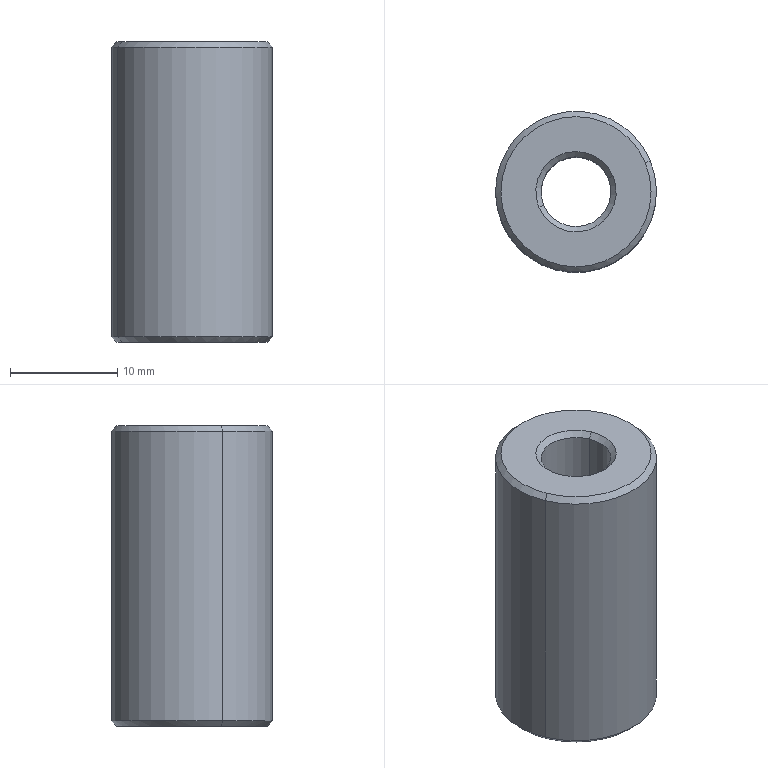Component | SolidWorks | WT-FLD-EJG-1212-00-024-1 | 1 solid | 14 faces | box 15 x 15 x 28 mm | volume 4002 mm3 | cone 8 | cylinder 4 | plane 2 | commonest cylinder face diameters 6.5 x2 15 x2 | material AISI 1045 Steel, cold drawn
build123d program:
from build123d import *

# Parameters (mm, degrees)
SKETCH1_R                  = 7.5
BOSS_EXTRUDE1_DEPTH        = 28
F_6_5_6_5_DIAMETER_HOLE1_D = 6.5
CHAMFER1_SIZE              = 0.5


with BuildPart() as part:
    # Sketch1 → Boss-Extrude1 (new body)
    with BuildSketch(Plane.XY):
        Circle(SKETCH1_R)
    extrude(amount=BOSS_EXTRUDE1_DEPTH)

    # 6.5 _6.5_ Diameter Hole1 (through all)
    with Locations(Plane.XY.offset(28)):
        with Locations((0, 0)):
            Hole(F_6_5_6_5_DIAMETER_HOLE1_D / 2)

    # Chamfer1
    chamfer1_edges = [part.edges().sort_by_distance(p)[0] for p in [
        (-7.5, 0, 0),
        (-7.5, 0, 28),
        (3.25, 0, 28),
        (3.25, 0, 0),
    ]]
    chamfer(chamfer1_edges, length=CHAMFER1_SIZE)


solid = part.part

# Placed as in the assembly
solid = solid.moved(Location((-97, -50, 60), (0, 0, 0)))
STEP:
#1=COLOUR_RGB('',0.7922,0.8196,0.9333);
#2=FILL_AREA_STYLE_COLOUR('',#1);
#3=FILL_AREA_STYLE('',(#2));
#4=SURFACE_STYLE_FILL_AREA(#3);
#5=SURFACE_SIDE_STYLE('',(#4));
#6=SURFACE_STYLE_USAGE(.BOTH.,#5);
#7=PRESENTATION_STYLE_ASSIGNMENT((#6));
#8=CARTESIAN_POINT('',(-3.701,-1.919,2.382));
#9=VERTEX_POINT('',#8);
#10=CARTESIAN_POINT('',(-3.937,-2.018,2.382));
#11=VERTEX_POINT('',#10);
#12=CARTESIAN_POINT('',(-3.819,-1.969,2.382));
#13=DIRECTION('',(0.,-0.,-1.));
#14=DIRECTION('',(-0.9237,-0.383,0.));
#15=AXIS2_PLACEMENT_3D('',#12,#13,#14);
#16=CIRCLE('',#15,0.128);
#17=EDGE_CURVE('',#9,#11,#16,.T.);
#18=ORIENTED_EDGE('',*,*,#17,.F.);
#19=CARTESIAN_POINT('',(-3.683,-1.912,2.362));
#20=VERTEX_POINT('',#19);
#21=CARTESIAN_POINT('',(-3.701,-1.919,2.382));
#22=DIRECTION('',(0.6532,0.2709,-0.7071));
#23=VECTOR('',#22,39.37);
#24=LINE('',#21,#23);
#25=EDGE_CURVE('',#9,#20,#24,.T.);
#26=ORIENTED_EDGE('',*,*,#25,.T.);
#27=CARTESIAN_POINT('',(-3.955,-2.025,2.362));
#28=VERTEX_POINT('',#27);
#29=CARTESIAN_POINT('',(-3.819,-1.969,2.362));
#30=DIRECTION('',(-0.,0.,1.));
#31=DIRECTION('',(-0.9237,-0.383,0.));
#32=AXIS2_PLACEMENT_3D('',#29,#30,#31);
#33=CIRCLE('',#32,0.1476);
#34=EDGE_CURVE('',#28,#20,#33,.T.);
#35=ORIENTED_EDGE('',*,*,#34,.F.);
#36=CARTESIAN_POINT('',(-3.937,-2.018,2.382));
#37=DIRECTION('',(-0.6532,-0.2709,-0.7071));
#38=VECTOR('',#37,39.37);
#39=LINE('',#36,#38);
#40=EDGE_CURVE('',#11,#28,#39,.T.);
#41=ORIENTED_EDGE('',*,*,#40,.F.);
#42=EDGE_LOOP('',(#18,#26,#35,#41));
#43=FACE_OUTER_BOUND('',#42,.T.);
#44=CARTESIAN_POINT('',(-3.819,-1.969,2.382));
#45=DIRECTION('',(0.,-0.,-1.));
#46=DIRECTION('',(-0.9237,-0.383,0.));
#47=AXIS2_PLACEMENT_3D('',#44,#45,#46);
#48=CONICAL_SURFACE('',#47,0.128,0.7854);
#49=ADVANCED_FACE('',(#43),#48,.F.);
#50=CARTESIAN_POINT('',(-4.073,-2.074,2.362));
#51=VERTEX_POINT('',#50);
#52=CARTESIAN_POINT('',(-3.564,-1.863,2.362));
#53=VERTEX_POINT('',#52);
#54=CARTESIAN_POINT('',(-3.819,-1.969,2.362));
#55=DIRECTION('',(0.,-0.,-1.));
#56=DIRECTION('',(-0.9237,-0.383,0.));
#57=AXIS2_PLACEMENT_3D('',#54,#55,#56);
#58=CIRCLE('',#57,0.2756);
#59=EDGE_CURVE('',#51,#53,#58,.T.);
#60=ORIENTED_EDGE('',*,*,#59,.F.);
#61=CARTESIAN_POINT('',(-4.092,-2.082,2.382));
#62=VERTEX_POINT('',#61);
#63=CARTESIAN_POINT('',(-4.073,-2.074,2.362));
#64=DIRECTION('',(-0.6532,-0.2709,0.7071));
#65=VECTOR('',#64,39.37);
#66=LINE('',#63,#65);
#67=EDGE_CURVE('',#51,#62,#66,.T.);
#68=ORIENTED_EDGE('',*,*,#67,.T.);
#69=CARTESIAN_POINT('',(-3.546,-1.855,2.382));
#70=VERTEX_POINT('',#69);
#71=CARTESIAN_POINT('',(-3.819,-1.969,2.382));
#72=DIRECTION('',(-0.,0.,1.));
#73=DIRECTION('',(-0.9237,-0.383,0.));
#74=AXIS2_PLACEMENT_3D('',#71,#72,#73);
#75=CIRCLE('',#74,0.2953);
#76=EDGE_CURVE('',#70,#62,#75,.T.);
#77=ORIENTED_EDGE('',*,*,#76,.F.);
#78=CARTESIAN_POINT('',(-3.564,-1.863,2.362));
#79=DIRECTION('',(0.6532,0.2709,0.7071));
#80=VECTOR('',#79,39.37);
#81=LINE('',#78,#80);
#82=EDGE_CURVE('',#53,#70,#81,.T.);
#83=ORIENTED_EDGE('',*,*,#82,.F.);
#84=EDGE_LOOP('',(#60,#68,#77,#83));
#85=FACE_OUTER_BOUND('',#84,.T.);
#86=CARTESIAN_POINT('',(-3.819,-1.969,2.362));
#87=DIRECTION('',(-0.,0.,1.));
#88=DIRECTION('',(0.9237,0.383,-0.));
#89=AXIS2_PLACEMENT_3D('',#86,#87,#88);
#90=CONICAL_SURFACE('',#89,0.2756,0.7854);
#91=ADVANCED_FACE('',(#85),#90,.T.);
#92=CARTESIAN_POINT('',(-3.937,-2.018,3.445));
#93=VERTEX_POINT('',#92);
#94=CARTESIAN_POINT('',(-3.701,-1.919,3.445));
#95=VERTEX_POINT('',#94);
#96=CARTESIAN_POINT('',(-3.819,-1.969,3.445));
#97=DIRECTION('',(-0.,0.,1.));
#98=DIRECTION('',(-0.9237,-0.383,0.));
#99=AXIS2_PLACEMENT_3D('',#96,#97,#98);
#100=CIRCLE('',#99,0.128);
#101=EDGE_CURVE('',#93,#95,#100,.T.);
#102=ORIENTED_EDGE('',*,*,#101,.F.);
#103=CARTESIAN_POINT('',(-3.955,-2.025,3.465));
#104=VERTEX_POINT('',#103);
#105=CARTESIAN_POINT('',(-3.955,-2.025,3.465));
#106=DIRECTION('',(-0.6532,-0.2709,0.7071));
#107=VECTOR('',#106,39.37);
#108=LINE('',#105,#107);
#109=EDGE_CURVE('',#93,#104,#108,.T.);
#110=ORIENTED_EDGE('',*,*,#109,.T.);
#111=CARTESIAN_POINT('',(-3.683,-1.912,3.465));
#112=VERTEX_POINT('',#111);
#113=CARTESIAN_POINT('',(-3.819,-1.969,3.465));
#114=DIRECTION('',(0.,-0.,-1.));
#115=DIRECTION('',(-0.9237,-0.383,0.));
#116=AXIS2_PLACEMENT_3D('',#113,#114,#115);
#117=CIRCLE('',#116,0.1476);
#118=EDGE_CURVE('',#112,#104,#117,.T.);
#119=ORIENTED_EDGE('',*,*,#118,.F.);
#120=CARTESIAN_POINT('',(-3.683,-1.912,3.465));
#121=DIRECTION('',(0.6532,0.2709,0.7071));
#122=VECTOR('',#121,39.37);
#123=LINE('',#120,#122);
#124=EDGE_CURVE('',#95,#112,#123,.T.);
#125=ORIENTED_EDGE('',*,*,#124,.F.);
#126=EDGE_LOOP('',(#102,#110,#119,#125));
#127=FACE_OUTER_BOUND('',#126,.T.);
#128=CARTESIAN_POINT('',(-3.819,-1.969,3.465));
#129=DIRECTION('',(-0.,0.,1.));
#130=DIRECTION('',(0.9237,0.383,0.));
#131=AXIS2_PLACEMENT_3D('',#128,#129,#130);
#132=CONICAL_SURFACE('',#131,0.1476,0.7854);
#133=ADVANCED_FACE('',(#127),#132,.F.);
#134=CARTESIAN_POINT('',(-3.564,-1.863,3.465));
#135=VERTEX_POINT('',#134);
#136=CARTESIAN_POINT('',(-4.073,-2.074,3.465));
#137=VERTEX_POINT('',#136);
#138=CARTESIAN_POINT('',(-3.819,-1.969,3.465));
#139=DIRECTION('',(-0.,0.,1.));
#140=DIRECTION('',(-0.9237,-0.383,0.));
#141=AXIS2_PLACEMENT_3D('',#138,#139,#140);
#142=CIRCLE('',#141,0.2756);
#143=EDGE_CURVE('',#135,#137,#142,.T.);
#144=ORIENTED_EDGE('',*,*,#143,.F.);
#145=CARTESIAN_POINT('',(-3.546,-1.855,3.445));
#146=VERTEX_POINT('',#145);
#147=CARTESIAN_POINT('',(-3.546,-1.855,3.445));
#148=DIRECTION('',(0.6532,0.2709,-0.7071));
#149=VECTOR('',#148,39.37);
#150=LINE('',#147,#149);
#151=EDGE_CURVE('',#135,#146,#150,.T.);
#152=ORIENTED_EDGE('',*,*,#151,.T.);
#153=CARTESIAN_POINT('',(-4.092,-2.082,3.445));
#154=VERTEX_POINT('',#153);
#155=CARTESIAN_POINT('',(-3.819,-1.969,3.445));
#156=DIRECTION('',(0.,-0.,-1.));
#157=DIRECTION('',(-0.9237,-0.383,0.));
#158=AXIS2_PLACEMENT_3D('',#155,#156,#157);
#159=CIRCLE('',#158,0.2953);
#160=EDGE_CURVE('',#154,#146,#159,.T.);
#161=ORIENTED_EDGE('',*,*,#160,.F.);
#162=CARTESIAN_POINT('',(-4.092,-2.082,3.445));
#163=DIRECTION('',(-0.6532,-0.2709,-0.7071));
#164=VECTOR('',#163,39.37);
#165=LINE('',#162,#164);
#166=EDGE_CURVE('',#137,#154,#165,.T.);
#167=ORIENTED_EDGE('',*,*,#166,.F.);
#168=EDGE_LOOP('',(#144,#152,#161,#167));
#169=FACE_OUTER_BOUND('',#168,.T.);
#170=CARTESIAN_POINT('',(-3.819,-1.969,3.445));
#171=DIRECTION('',(0.,-0.,-1.));
#172=DIRECTION('',(-0.9237,-0.383,0.));
#173=AXIS2_PLACEMENT_3D('',#170,#171,#172);
#174=CONICAL_SURFACE('',#173,0.2953,0.7854);
#175=ADVANCED_FACE('',(#169),#174,.T.);
#176=ORIENTED_EDGE('',*,*,#101,.T.);
#177=CARTESIAN_POINT('',(-3.701,-1.919,2.362));
#178=DIRECTION('',(0.,-0.,-1.));
#179=VECTOR('',#178,39.37);
#180=LINE('',#177,#179);
#181=EDGE_CURVE('',#95,#9,#180,.T.);
#182=ORIENTED_EDGE('',*,*,#181,.T.);
#183=ORIENTED_EDGE('',*,*,#17,.T.);
#184=CARTESIAN_POINT('',(-3.937,-2.018,2.362));
#185=DIRECTION('',(0.,-0.,-1.));
#186=VECTOR('',#185,39.37);
#187=LINE('',#184,#186);
#188=EDGE_CURVE('',#93,#11,#187,.T.);
#189=ORIENTED_EDGE('',*,*,#188,.F.);
#190=EDGE_LOOP('',(#176,#182,#183,#189));
#191=FACE_OUTER_BOUND('',#190,.T.);
#192=CARTESIAN_POINT('',(-3.819,-1.969,2.362));
#193=DIRECTION('',(0.,-0.,-1.));
#194=DIRECTION('',(-0.9237,-0.383,0.));
#195=AXIS2_PLACEMENT_3D('',#192,#193,#194);
#196=CYLINDRICAL_SURFACE('',#195,0.128);
#197=ADVANCED_FACE('',(#191),#196,.F.);
#198=ORIENTED_EDGE('',*,*,#76,.T.);
#199=CARTESIAN_POINT('',(-4.092,-2.082,2.362));
#200=DIRECTION('',(-0.,0.,1.));
#201=VECTOR('',#200,39.37);
#202=LINE('',#199,#201);
#203=EDGE_CURVE('',#62,#154,#202,.T.);
#204=ORIENTED_EDGE('',*,*,#203,.T.);
#205=ORIENTED_EDGE('',*,*,#160,.T.);
#206=CARTESIAN_POINT('',(-3.546,-1.855,2.362));
#207=DIRECTION('',(-0.,0.,1.));
#208=VECTOR('',#207,39.37);
#209=LINE('',#206,#208);
#210=EDGE_CURVE('',#70,#146,#209,.T.);
#211=ORIENTED_EDGE('',*,*,#210,.F.);
#212=EDGE_LOOP('',(#198,#204,#205,#211));
#213=FACE_OUTER_BOUND('',#212,.T.);
#214=CARTESIAN_POINT('',(-3.819,-1.969,2.362));
#215=DIRECTION('',(-0.,0.,1.));
#216=DIRECTION('',(0.9237,0.383,-0.));
#217=AXIS2_PLACEMENT_3D('',#214,#215,#216);
#218=CYLINDRICAL_SURFACE('',#217,0.2953);
#219=ADVANCED_FACE('',(#213),#218,.T.);
#220=ORIENTED_EDGE('',*,*,#203,.F.);
#221=CARTESIAN_POINT('',(-3.819,-1.969,2.382));
#222=DIRECTION('',(-0.,0.,1.));
#223=DIRECTION('',(-0.9237,-0.383,0.));
#224=AXIS2_PLACEMENT_3D('',#221,#222,#223);
#225=CIRCLE('',#224,0.2953);
#226=EDGE_CURVE('',#62,#70,#225,.T.);
#227=ORIENTED_EDGE('',*,*,#226,.T.);
#228=ORIENTED_EDGE('',*,*,#210,.T.);
#229=CARTESIAN_POINT('',(-3.819,-1.969,3.445));
#230=DIRECTION('',(0.,-0.,-1.));
#231=DIRECTION('',(-0.9237,-0.383,0.));
#232=AXIS2_PLACEMENT_3D('',#229,#230,#231);
#233=CIRCLE('',#232,0.2953);
#234=EDGE_CURVE('',#146,#154,#233,.T.);
#235=ORIENTED_EDGE('',*,*,#234,.T.);
#236=EDGE_LOOP('',(#220,#227,#228,#235));
#237=FACE_OUTER_BOUND('',#236,.T.);
#238=CARTESIAN_POINT('',(-3.819,-1.969,2.362));
#239=DIRECTION('',(-0.,0.,1.));
#240=DIRECTION('',(0.9237,0.383,-0.));
#241=AXIS2_PLACEMENT_3D('',#238,#239,#240);
#242=CYLINDRICAL_SURFACE('',#241,0.2953);
#243=ADVANCED_FACE('',(#237),#242,.T.);
#244=CARTESIAN_POINT('',(-3.819,-1.969,2.362));
#245=DIRECTION('',(0.,-0.,-1.));
#246=DIRECTION('',(-0.9237,-0.383,0.));
#247=AXIS2_PLACEMENT_3D('',#244,#245,#246);
#248=CIRCLE('',#247,0.2756);
#249=EDGE_CURVE('',#53,#51,#248,.T.);
#250=ORIENTED_EDGE('',*,*,#249,.T.);
#251=ORIENTED_EDGE('',*,*,#59,.T.);
#252=EDGE_LOOP('',(#250,#251));
#253=FACE_OUTER_BOUND('',#252,.T.);
#254=ORIENTED_EDGE('',*,*,#34,.T.);
#255=CARTESIAN_POINT('',(-3.819,-1.969,2.362));
#256=DIRECTION('',(-0.,0.,1.));
#257=DIRECTION('',(-0.9237,-0.383,0.));
#258=AXIS2_PLACEMENT_3D('',#255,#256,#257);
#259=CIRCLE('',#258,0.1476);
#260=EDGE_CURVE('',#20,#28,#259,.T.);
#261=ORIENTED_EDGE('',*,*,#260,.T.);
#262=EDGE_LOOP('',(#254,#261));
#263=FACE_BOUND('',#262,.T.);
#264=CARTESIAN_POINT('',(-3.819,-1.969,2.362));
#265=DIRECTION('',(0.,-0.,-1.));
#266=DIRECTION('',(-0.9237,-0.383,0.));
#267=AXIS2_PLACEMENT_3D('',#264,#265,#266);
#268=PLANE('',#267);
#269=ADVANCED_FACE('',(#253,#263),#268,.T.);
#270=CARTESIAN_POINT('',(-3.819,-1.969,3.465));
#271=DIRECTION('',(-0.,0.,1.));
#272=DIRECTION('',(-0.9237,-0.383,0.));
#273=AXIS2_PLACEMENT_3D('',#270,#271,#272);
#274=CIRCLE('',#273,0.2756);
#275=EDGE_CURVE('',#137,#135,#274,.T.);
#276=ORIENTED_EDGE('',*,*,#275,.T.);
#277=ORIENTED_EDGE('',*,*,#143,.T.);
#278=EDGE_LOOP('',(#276,#277));
#279=FACE_OUTER_BOUND('',#278,.T.);
#280=ORIENTED_EDGE('',*,*,#118,.T.);
#281=CARTESIAN_POINT('',(-3.819,-1.969,3.465));
#282=DIRECTION('',(0.,-0.,-1.));
#283=DIRECTION('',(-0.9237,-0.383,0.));
#284=AXIS2_PLACEMENT_3D('',#281,#282,#283);
#285=CIRCLE('',#284,0.1476);
#286=EDGE_CURVE('',#104,#112,#285,.T.);
#287=ORIENTED_EDGE('',*,*,#286,.T.);
#288=EDGE_LOOP('',(#280,#287));
#289=FACE_BOUND('',#288,.T.);
#290=CARTESIAN_POINT('',(-3.819,-1.969,3.465));
#291=DIRECTION('',(0.,-0.,-1.));
#292=DIRECTION('',(-0.9237,-0.383,0.));
#293=AXIS2_PLACEMENT_3D('',#290,#291,#292);
#294=PLANE('',#293);
#295=ADVANCED_FACE('',(#279,#289),#294,.F.);
#296=ORIENTED_EDGE('',*,*,#181,.F.);
#297=CARTESIAN_POINT('',(-3.819,-1.969,3.445));
#298=DIRECTION('',(-0.,0.,1.));
#299=DIRECTION('',(-0.9237,-0.383,0.));
#300=AXIS2_PLACEMENT_3D('',#297,#298,#299);
#301=CIRCLE('',#300,0.128);
#302=EDGE_CURVE('',#95,#93,#301,.T.);
#303=ORIENTED_EDGE('',*,*,#302,.T.);
#304=ORIENTED_EDGE('',*,*,#188,.T.);
#305=CARTESIAN_POINT('',(-3.819,-1.969,2.382));
#306=DIRECTION('',(0.,-0.,-1.));
#307=DIRECTION('',(-0.9237,-0.383,0.));
#308=AXIS2_PLACEMENT_3D('',#305,#306,#307);
#309=CIRCLE('',#308,0.128);
#310=EDGE_CURVE('',#11,#9,#309,.T.);
#311=ORIENTED_EDGE('',*,*,#310,.T.);
#312=EDGE_LOOP('',(#296,#303,#304,#311));
#313=FACE_OUTER_BOUND('',#312,.T.);
#314=CARTESIAN_POINT('',(-3.819,-1.969,2.362));
#315=DIRECTION('',(0.,-0.,-1.));
#316=DIRECTION('',(-0.9237,-0.383,0.));
#317=AXIS2_PLACEMENT_3D('',#314,#315,#316);
#318=CYLINDRICAL_SURFACE('',#317,0.128);
#319=ADVANCED_FACE('',(#313),#318,.F.);
#320=ORIENTED_EDGE('',*,*,#151,.F.);
#321=ORIENTED_EDGE('',*,*,#275,.F.);
#322=ORIENTED_EDGE('',*,*,#166,.T.);
#323=ORIENTED_EDGE('',*,*,#234,.F.);
#324=EDGE_LOOP('',(#320,#321,#322,#323));
#325=FACE_OUTER_BOUND('',#324,.T.);
#326=CARTESIAN_POINT('',(-3.819,-1.969,3.445));
#327=DIRECTION('',(0.,-0.,-1.));
#328=DIRECTION('',(-0.9237,-0.383,0.));
#329=AXIS2_PLACEMENT_3D('',#326,#327,#328);
#330=CONICAL_SURFACE('',#329,0.2953,0.7854);
#331=ADVANCED_FACE('',(#325),#330,.T.);
#332=ORIENTED_EDGE('',*,*,#109,.F.);
#333=ORIENTED_EDGE('',*,*,#302,.F.);
#334=ORIENTED_EDGE('',*,*,#124,.T.);
#335=ORIENTED_EDGE('',*,*,#286,.F.);
#336=EDGE_LOOP('',(#332,#333,#334,#335));
#337=FACE_OUTER_BOUND('',#336,.T.);
#338=CARTESIAN_POINT('',(-3.819,-1.969,3.465));
#339=DIRECTION('',(-0.,0.,1.));
#340=DIRECTION('',(0.9237,0.383,0.));
#341=AXIS2_PLACEMENT_3D('',#338,#339,#340);
#342=CONICAL_SURFACE('',#341,0.1476,0.7854);
#343=ADVANCED_FACE('',(#337),#342,.F.);
#344=ORIENTED_EDGE('',*,*,#67,.F.);
#345=ORIENTED_EDGE('',*,*,#249,.F.);
#346=ORIENTED_EDGE('',*,*,#82,.T.);
#347=ORIENTED_EDGE('',*,*,#226,.F.);
#348=EDGE_LOOP('',(#344,#345,#346,#347));
#349=FACE_OUTER_BOUND('',#348,.T.);
#350=CARTESIAN_POINT('',(-3.819,-1.969,2.362));
#351=DIRECTION('',(-0.,0.,1.));
#352=DIRECTION('',(0.9237,0.383,-0.));
#353=AXIS2_PLACEMENT_3D('',#350,#351,#352);
#354=CONICAL_SURFACE('',#353,0.2756,0.7854);
#355=ADVANCED_FACE('',(#349),#354,.T.);
#356=ORIENTED_EDGE('',*,*,#25,.F.);
#357=ORIENTED_EDGE('',*,*,#310,.F.);
#358=ORIENTED_EDGE('',*,*,#40,.T.);
#359=ORIENTED_EDGE('',*,*,#260,.F.);
#360=EDGE_LOOP('',(#356,#357,#358,#359));
#361=FACE_OUTER_BOUND('',#360,.T.);
#362=CARTESIAN_POINT('',(-3.819,-1.969,2.382));
#363=DIRECTION('',(0.,-0.,-1.));
#364=DIRECTION('',(-0.9237,-0.383,0.));
#365=AXIS2_PLACEMENT_3D('',#362,#363,#364);
#366=CONICAL_SURFACE('',#365,0.128,0.7854);
#367=ADVANCED_FACE('',(#361),#366,.F.);
#368=CLOSED_SHELL('',(#49,#91,#133,#175,#197,#219,#243,#269,#295,#319,#331,#343,#355,#367));
#369=MANIFOLD_SOLID_BREP('',#368);
#370=STYLED_ITEM('',(#7),#369);
#371=PRESENTATION_LAYER_ASSIGNMENT('','',(#370));
#372=CARTESIAN_POINT('',(0.,0.,0.));
#373=DIRECTION('',(0.,0.,1.));
#374=DIRECTION('',(1.,0.,0.));
#375=AXIS2_PLACEMENT_3D('',#372,#373,#374);
#376=(LENGTH_UNIT()NAMED_UNIT(*)SI_UNIT($,.METRE.));
#377=LENGTH_MEASURE_WITH_UNIT(LENGTH_MEASURE(0.0254),#376);
#378=DIMENSIONAL_EXPONENTS(1.,0.,0.,0.,0.,0.,0.);
#379=(CONVERSION_BASED_UNIT('',#377)LENGTH_UNIT()NAMED_UNIT(#378));
#380=UNCERTAINTY_MEASURE_WITH_UNIT(LENGTH_MEASURE(0.00001),#379,'','');
#381=(NAMED_UNIT(*)PLANE_ANGLE_UNIT()SI_UNIT($,.RADIAN.));
#382=(NAMED_UNIT(*)SI_UNIT($,.STERADIAN.)SOLID_ANGLE_UNIT());
#383=(GEOMETRIC_REPRESENTATION_CONTEXT(3)GLOBAL_UNCERTAINTY_ASSIGNED_CONTEXT((#380))GLOBAL_UNIT_ASSIGNED_CONTEXT((#379,#381,#382))REPRESENTATION_CONTEXT('',''));
#384=ADVANCED_BREP_SHAPE_REPRESENTATION('',(#369,#375),#383);
#385=(LENGTH_UNIT()NAMED_UNIT(*)SI_UNIT($,.METRE.));
#386=LENGTH_MEASURE_WITH_UNIT(LENGTH_MEASURE(0.0254),#385);
#387=DIMENSIONAL_EXPONENTS(1.,0.,0.,0.,0.,0.,0.);
#388=(CONVERSION_BASED_UNIT('',#386)LENGTH_UNIT()NAMED_UNIT(#387));
#389=UNCERTAINTY_MEASURE_WITH_UNIT(LENGTH_MEASURE(0.00001),#388,'','');
#390=(NAMED_UNIT(*)PLANE_ANGLE_UNIT()SI_UNIT($,.RADIAN.));
#391=(NAMED_UNIT(*)SI_UNIT($,.STERADIAN.)SOLID_ANGLE_UNIT());
#392=(GEOMETRIC_REPRESENTATION_CONTEXT(3)GLOBAL_UNCERTAINTY_ASSIGNED_CONTEXT((#389))GLOBAL_UNIT_ASSIGNED_CONTEXT((#388,#390,#391))REPRESENTATION_CONTEXT('',''));
#393=MECHANICAL_DESIGN_GEOMETRIC_PRESENTATION_REPRESENTATION('',(#370),#392);